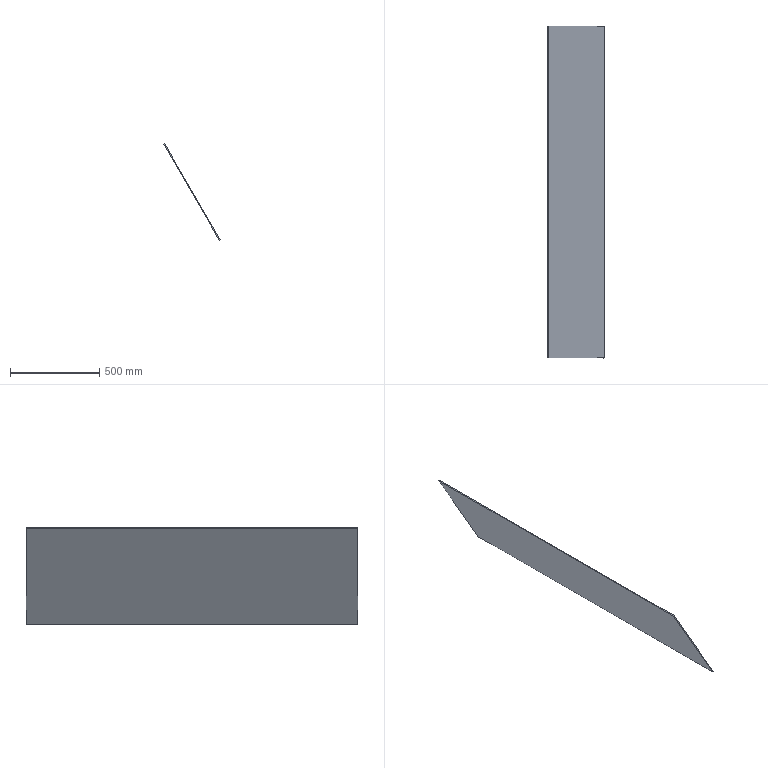Component | SolidWorks | FrontDoorAssembly-1_Glass-1 | 1 solid | 6 faces | box 314.33 x 1860 x 539.44 mm | volume 5766000 mm3 | plane 6 | material Malleable Cast Iron
STEP:
#1=COLOUR_RGB('',0.7922,0.8196,0.9333);
#2=FILL_AREA_STYLE_COLOUR('',#1);
#3=FILL_AREA_STYLE('',(#2));
#4=SURFACE_STYLE_FILL_AREA(#3);
#5=SURFACE_SIDE_STYLE('',(#4));
#6=SURFACE_STYLE_USAGE(.BOTH.,#5);
#7=PRESENTATION_STYLE_ASSIGNMENT((#6));
#8=CARTESIAN_POINT('',(10.553,73.089,18.865));
#9=VERTEX_POINT('',#8);
#10=CARTESIAN_POINT('',(10.553,-0.1394,18.865));
#11=VERTEX_POINT('',#10);
#12=CARTESIAN_POINT('',(10.553,73.089,18.865));
#13=DIRECTION('',(0.,-1.,-0.));
#14=VECTOR('',#13,39.37);
#15=LINE('',#12,#14);
#16=EDGE_CURVE('',#9,#11,#15,.T.);
#17=ORIENTED_EDGE('',*,*,#16,.F.);
#18=CARTESIAN_POINT('',(10.723,73.089,18.963));
#19=VERTEX_POINT('',#18);
#20=CARTESIAN_POINT('',(10.723,73.089,18.963));
#21=DIRECTION('',(-0.866,-0.,-0.5));
#22=VECTOR('',#21,39.37);
#23=LINE('',#20,#22);
#24=EDGE_CURVE('',#19,#9,#23,.T.);
#25=ORIENTED_EDGE('',*,*,#24,.F.);
#26=CARTESIAN_POINT('',(10.723,-0.1394,18.963));
#27=VERTEX_POINT('',#26);
#28=CARTESIAN_POINT('',(10.723,73.089,18.963));
#29=DIRECTION('',(0.,-1.,-0.));
#30=VECTOR('',#29,39.37);
#31=LINE('',#28,#30);
#32=EDGE_CURVE('',#19,#27,#31,.T.);
#33=ORIENTED_EDGE('',*,*,#32,.T.);
#34=CARTESIAN_POINT('',(10.723,-0.1394,18.963));
#35=DIRECTION('',(-0.866,-0.,-0.5));
#36=VECTOR('',#35,39.37);
#37=LINE('',#34,#36);
#38=EDGE_CURVE('',#27,#11,#37,.T.);
#39=ORIENTED_EDGE('',*,*,#38,.T.);
#40=EDGE_LOOP('',(#17,#25,#33,#39));
#41=FACE_OUTER_BOUND('',#40,.T.);
#42=CARTESIAN_POINT('',(10.723,73.089,18.963));
#43=DIRECTION('',(0.5,0.,-0.866));
#44=DIRECTION('',(0.,-1.,-0.));
#45=AXIS2_PLACEMENT_3D('',#42,#43,#44);
#46=PLANE('',#45);
#47=ADVANCED_FACE('',(#41),#46,.T.);
#48=CARTESIAN_POINT('',(-1.652,73.089,40.004));
#49=VERTEX_POINT('',#48);
#50=CARTESIAN_POINT('',(10.553,73.089,18.865));
#51=DIRECTION('',(0.5,0.,-0.866));
#52=VECTOR('',#51,39.37);
#53=LINE('',#50,#52);
#54=EDGE_CURVE('',#49,#9,#53,.T.);
#55=ORIENTED_EDGE('',*,*,#54,.F.);
#56=CARTESIAN_POINT('',(-1.481,73.089,40.102));
#57=VERTEX_POINT('',#56);
#58=CARTESIAN_POINT('',(-1.481,73.089,40.102));
#59=DIRECTION('',(-0.866,-0.,-0.5));
#60=VECTOR('',#59,39.37);
#61=LINE('',#58,#60);
#62=EDGE_CURVE('',#57,#49,#61,.T.);
#63=ORIENTED_EDGE('',*,*,#62,.F.);
#64=CARTESIAN_POINT('',(10.723,73.089,18.963));
#65=DIRECTION('',(0.5,0.,-0.866));
#66=VECTOR('',#65,39.37);
#67=LINE('',#64,#66);
#68=EDGE_CURVE('',#57,#19,#67,.T.);
#69=ORIENTED_EDGE('',*,*,#68,.T.);
#70=ORIENTED_EDGE('',*,*,#24,.T.);
#71=EDGE_LOOP('',(#55,#63,#69,#70));
#72=FACE_OUTER_BOUND('',#71,.T.);
#73=CARTESIAN_POINT('',(10.723,73.089,18.963));
#74=DIRECTION('',(-0.,1.,0.));
#75=DIRECTION('',(-0.866,-0.,-0.5));
#76=AXIS2_PLACEMENT_3D('',#73,#74,#75);
#77=PLANE('',#76);
#78=ADVANCED_FACE('',(#72),#77,.T.);
#79=CARTESIAN_POINT('',(-1.652,-0.1394,40.004));
#80=VERTEX_POINT('',#79);
#81=CARTESIAN_POINT('',(-1.652,73.089,40.004));
#82=DIRECTION('',(-0.,1.,0.));
#83=VECTOR('',#82,39.37);
#84=LINE('',#81,#83);
#85=EDGE_CURVE('',#80,#49,#84,.T.);
#86=ORIENTED_EDGE('',*,*,#85,.F.);
#87=CARTESIAN_POINT('',(-1.481,-0.1394,40.102));
#88=VERTEX_POINT('',#87);
#89=CARTESIAN_POINT('',(-1.481,-0.1394,40.102));
#90=DIRECTION('',(-0.866,-0.,-0.5));
#91=VECTOR('',#90,39.37);
#92=LINE('',#89,#91);
#93=EDGE_CURVE('',#88,#80,#92,.T.);
#94=ORIENTED_EDGE('',*,*,#93,.F.);
#95=CARTESIAN_POINT('',(-1.481,73.089,40.102));
#96=DIRECTION('',(-0.,1.,0.));
#97=VECTOR('',#96,39.37);
#98=LINE('',#95,#97);
#99=EDGE_CURVE('',#88,#57,#98,.T.);
#100=ORIENTED_EDGE('',*,*,#99,.T.);
#101=ORIENTED_EDGE('',*,*,#62,.T.);
#102=EDGE_LOOP('',(#86,#94,#100,#101));
#103=FACE_OUTER_BOUND('',#102,.T.);
#104=CARTESIAN_POINT('',(-1.481,73.089,40.102));
#105=DIRECTION('',(-0.5,-0.,0.866));
#106=DIRECTION('',(-0.,1.,0.));
#107=AXIS2_PLACEMENT_3D('',#104,#105,#106);
#108=PLANE('',#107);
#109=ADVANCED_FACE('',(#103),#108,.T.);
#110=CARTESIAN_POINT('',(10.553,-0.1394,18.865));
#111=DIRECTION('',(-0.5,-0.,0.866));
#112=VECTOR('',#111,39.37);
#113=LINE('',#110,#112);
#114=EDGE_CURVE('',#11,#80,#113,.T.);
#115=ORIENTED_EDGE('',*,*,#114,.F.);
#116=ORIENTED_EDGE('',*,*,#38,.F.);
#117=CARTESIAN_POINT('',(10.723,-0.1394,18.963));
#118=DIRECTION('',(-0.5,-0.,0.866));
#119=VECTOR('',#118,39.37);
#120=LINE('',#117,#119);
#121=EDGE_CURVE('',#27,#88,#120,.T.);
#122=ORIENTED_EDGE('',*,*,#121,.T.);
#123=ORIENTED_EDGE('',*,*,#93,.T.);
#124=EDGE_LOOP('',(#115,#116,#122,#123));
#125=FACE_OUTER_BOUND('',#124,.T.);
#126=CARTESIAN_POINT('',(10.723,-0.1394,18.963));
#127=DIRECTION('',(0.,-1.,-0.));
#128=DIRECTION('',(0.866,0.,0.5));
#129=AXIS2_PLACEMENT_3D('',#126,#127,#128);
#130=PLANE('',#129);
#131=ADVANCED_FACE('',(#125),#130,.T.);
#132=ORIENTED_EDGE('',*,*,#32,.F.);
#133=ORIENTED_EDGE('',*,*,#68,.F.);
#134=ORIENTED_EDGE('',*,*,#99,.F.);
#135=ORIENTED_EDGE('',*,*,#121,.F.);
#136=EDGE_LOOP('',(#132,#133,#134,#135));
#137=FACE_OUTER_BOUND('',#136,.T.);
#138=CARTESIAN_POINT('',(8.088,71.204,23.528));
#139=DIRECTION('',(-0.866,-0.,-0.5));
#140=DIRECTION('',(-0.5,-0.,0.866));
#141=AXIS2_PLACEMENT_3D('',#138,#139,#140);
#142=PLANE('',#141);
#143=ADVANCED_FACE('',(#137),#142,.F.);
#144=ORIENTED_EDGE('',*,*,#16,.T.);
#145=ORIENTED_EDGE('',*,*,#114,.T.);
#146=ORIENTED_EDGE('',*,*,#85,.T.);
#147=ORIENTED_EDGE('',*,*,#54,.T.);
#148=EDGE_LOOP('',(#144,#145,#146,#147));
#149=FACE_OUTER_BOUND('',#148,.T.);
#150=CARTESIAN_POINT('',(7.917,71.204,23.43));
#151=DIRECTION('',(-0.866,-0.,-0.5));
#152=DIRECTION('',(-0.5,-0.,0.866));
#153=AXIS2_PLACEMENT_3D('',#150,#151,#152);
#154=PLANE('',#153);
#155=ADVANCED_FACE('',(#149),#154,.T.);
#156=CLOSED_SHELL('',(#47,#78,#109,#131,#143,#155));
#157=MANIFOLD_SOLID_BREP('',#156);
#158=STYLED_ITEM('',(#7),#157);
#159=(LENGTH_UNIT()NAMED_UNIT(*)SI_UNIT($,.METRE.));
#160=LENGTH_MEASURE_WITH_UNIT(LENGTH_MEASURE(0.0254),#159);
#161=DIMENSIONAL_EXPONENTS(1.,0.,0.,0.,0.,0.,0.);
#162=(CONVERSION_BASED_UNIT('',#160)LENGTH_UNIT()NAMED_UNIT(#161));
#163=UNCERTAINTY_MEASURE_WITH_UNIT(LENGTH_MEASURE(0.00001),#162,'','');
#164=(NAMED_UNIT(*)PLANE_ANGLE_UNIT()SI_UNIT($,.RADIAN.));
#165=(NAMED_UNIT(*)SI_UNIT($,.STERADIAN.)SOLID_ANGLE_UNIT());
#166=(GEOMETRIC_REPRESENTATION_CONTEXT(3)GLOBAL_UNCERTAINTY_ASSIGNED_CONTEXT((#163))GLOBAL_UNIT_ASSIGNED_CONTEXT((#162,#164,#165))REPRESENTATION_CONTEXT('',''));
#167=MECHANICAL_DESIGN_GEOMETRIC_PRESENTATION_REPRESENTATION('',(#158),#166);
#168=CARTESIAN_POINT('',(0.,0.,0.));
#169=DIRECTION('',(0.,0.,1.));
#170=DIRECTION('',(1.,0.,0.));
#171=AXIS2_PLACEMENT_3D('',#168,#169,#170);
#172=(LENGTH_UNIT()NAMED_UNIT(*)SI_UNIT($,.METRE.));
#173=LENGTH_MEASURE_WITH_UNIT(LENGTH_MEASURE(0.0254),#172);
#174=DIMENSIONAL_EXPONENTS(1.,0.,0.,0.,0.,0.,0.);
#175=(CONVERSION_BASED_UNIT('',#173)LENGTH_UNIT()NAMED_UNIT(#174));
#176=UNCERTAINTY_MEASURE_WITH_UNIT(LENGTH_MEASURE(0.00001),#175,'','');
#177=(NAMED_UNIT(*)PLANE_ANGLE_UNIT()SI_UNIT($,.RADIAN.));
#178=(NAMED_UNIT(*)SI_UNIT($,.STERADIAN.)SOLID_ANGLE_UNIT());
#179=(GEOMETRIC_REPRESENTATION_CONTEXT(3)GLOBAL_UNCERTAINTY_ASSIGNED_CONTEXT((#176))GLOBAL_UNIT_ASSIGNED_CONTEXT((#175,#177,#178))REPRESENTATION_CONTEXT('',''));
#180=ADVANCED_BREP_SHAPE_REPRESENTATION('',(#157,#171),#179);
#181=PRESENTATION_LAYER_ASSIGNMENT('','',(#158));